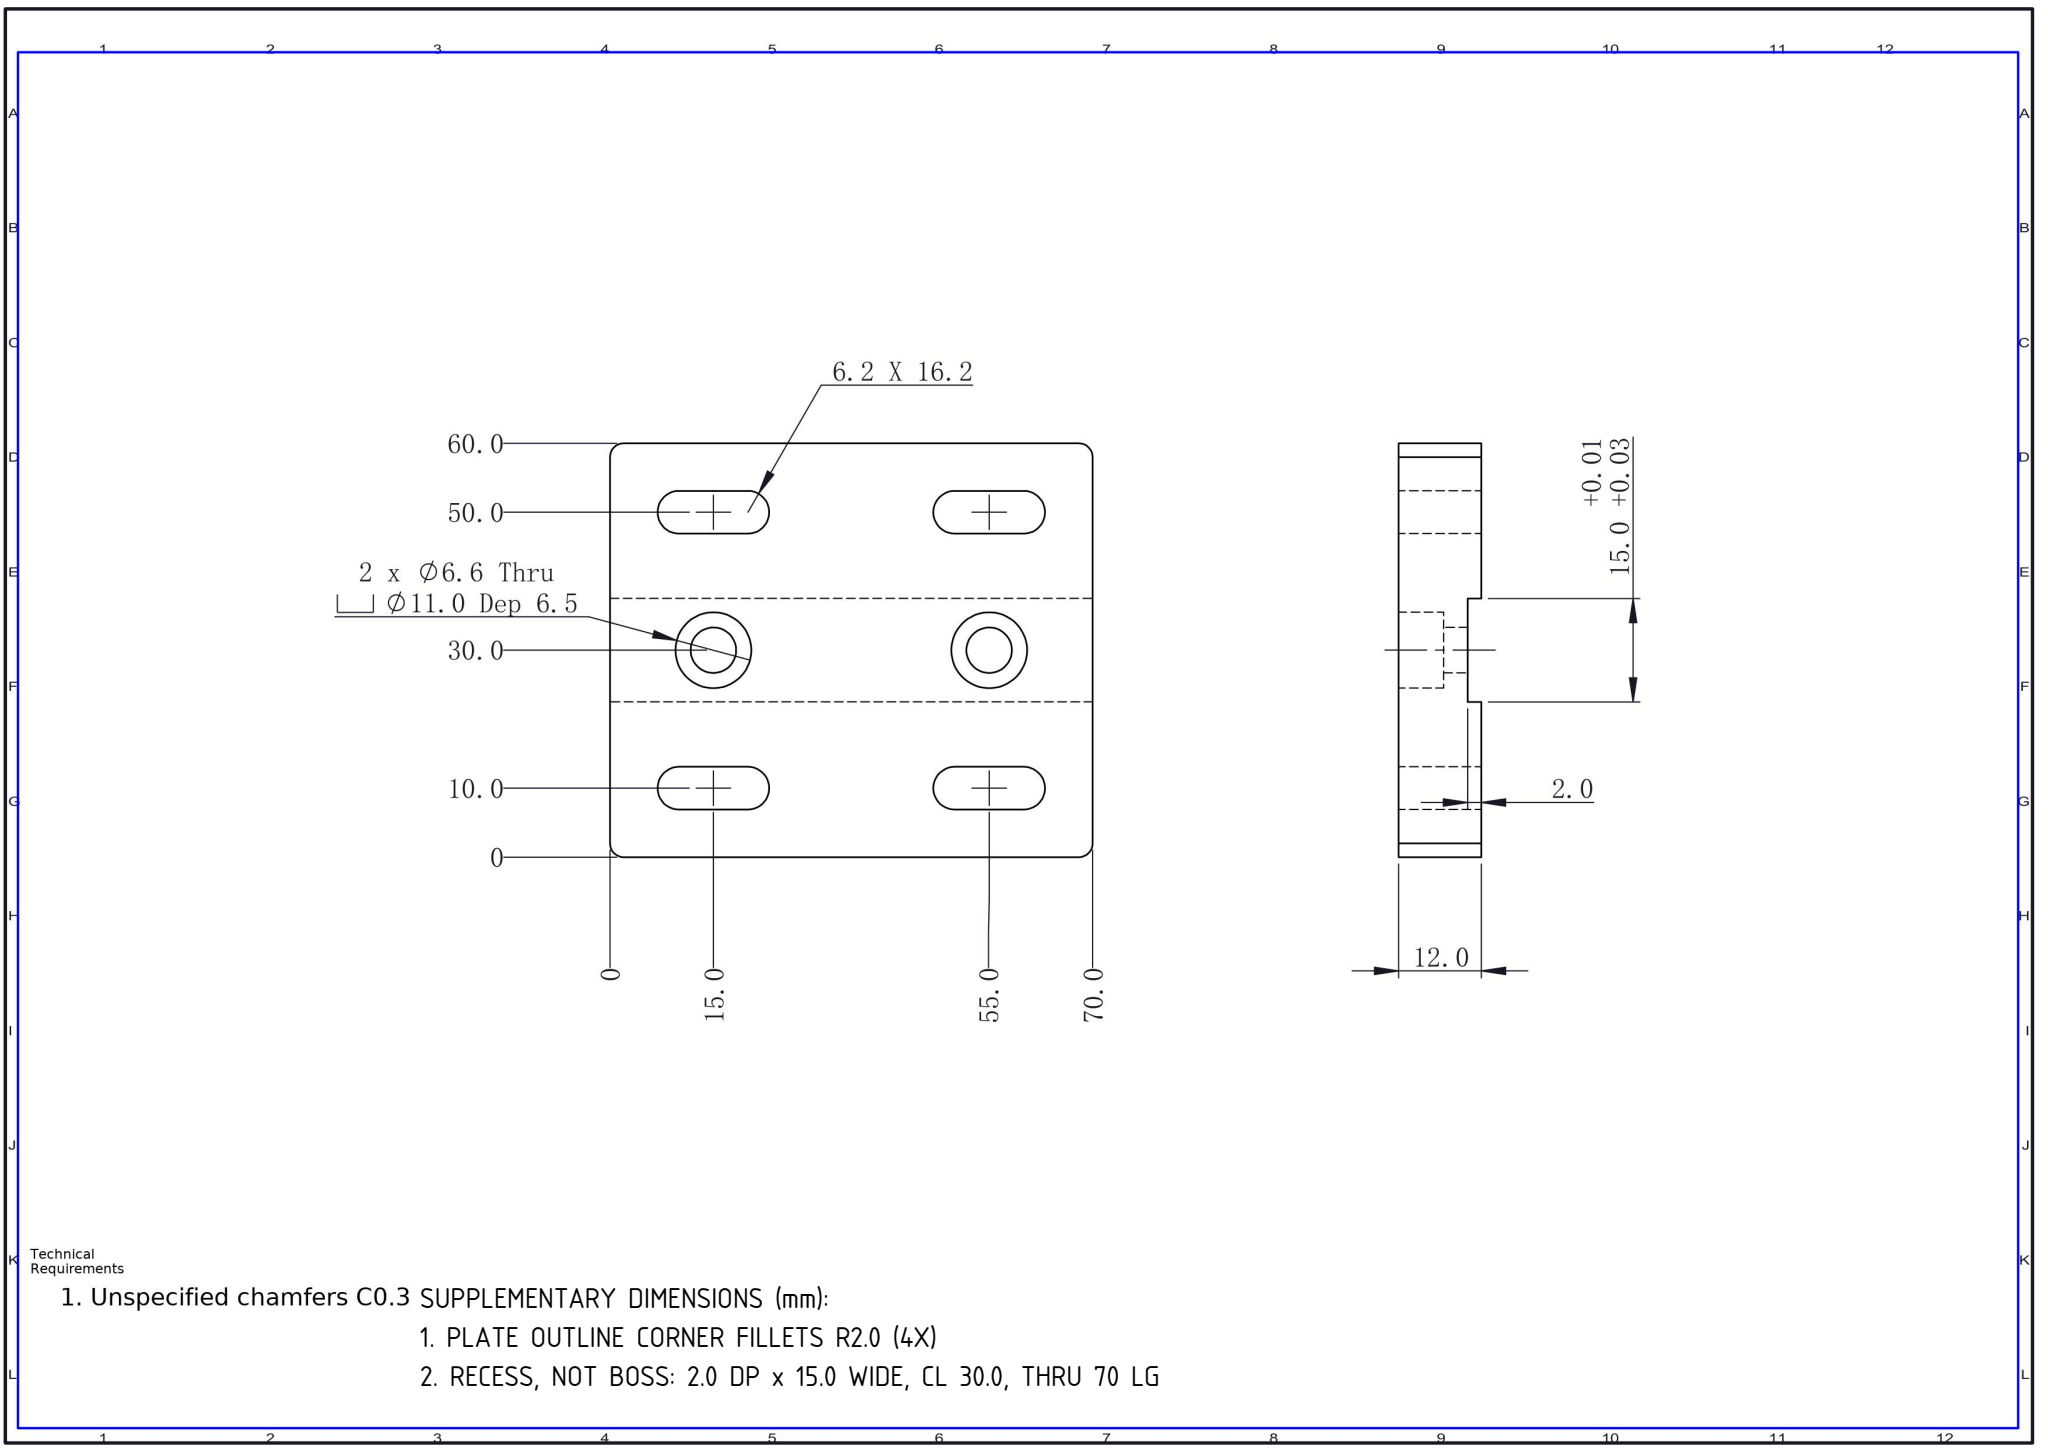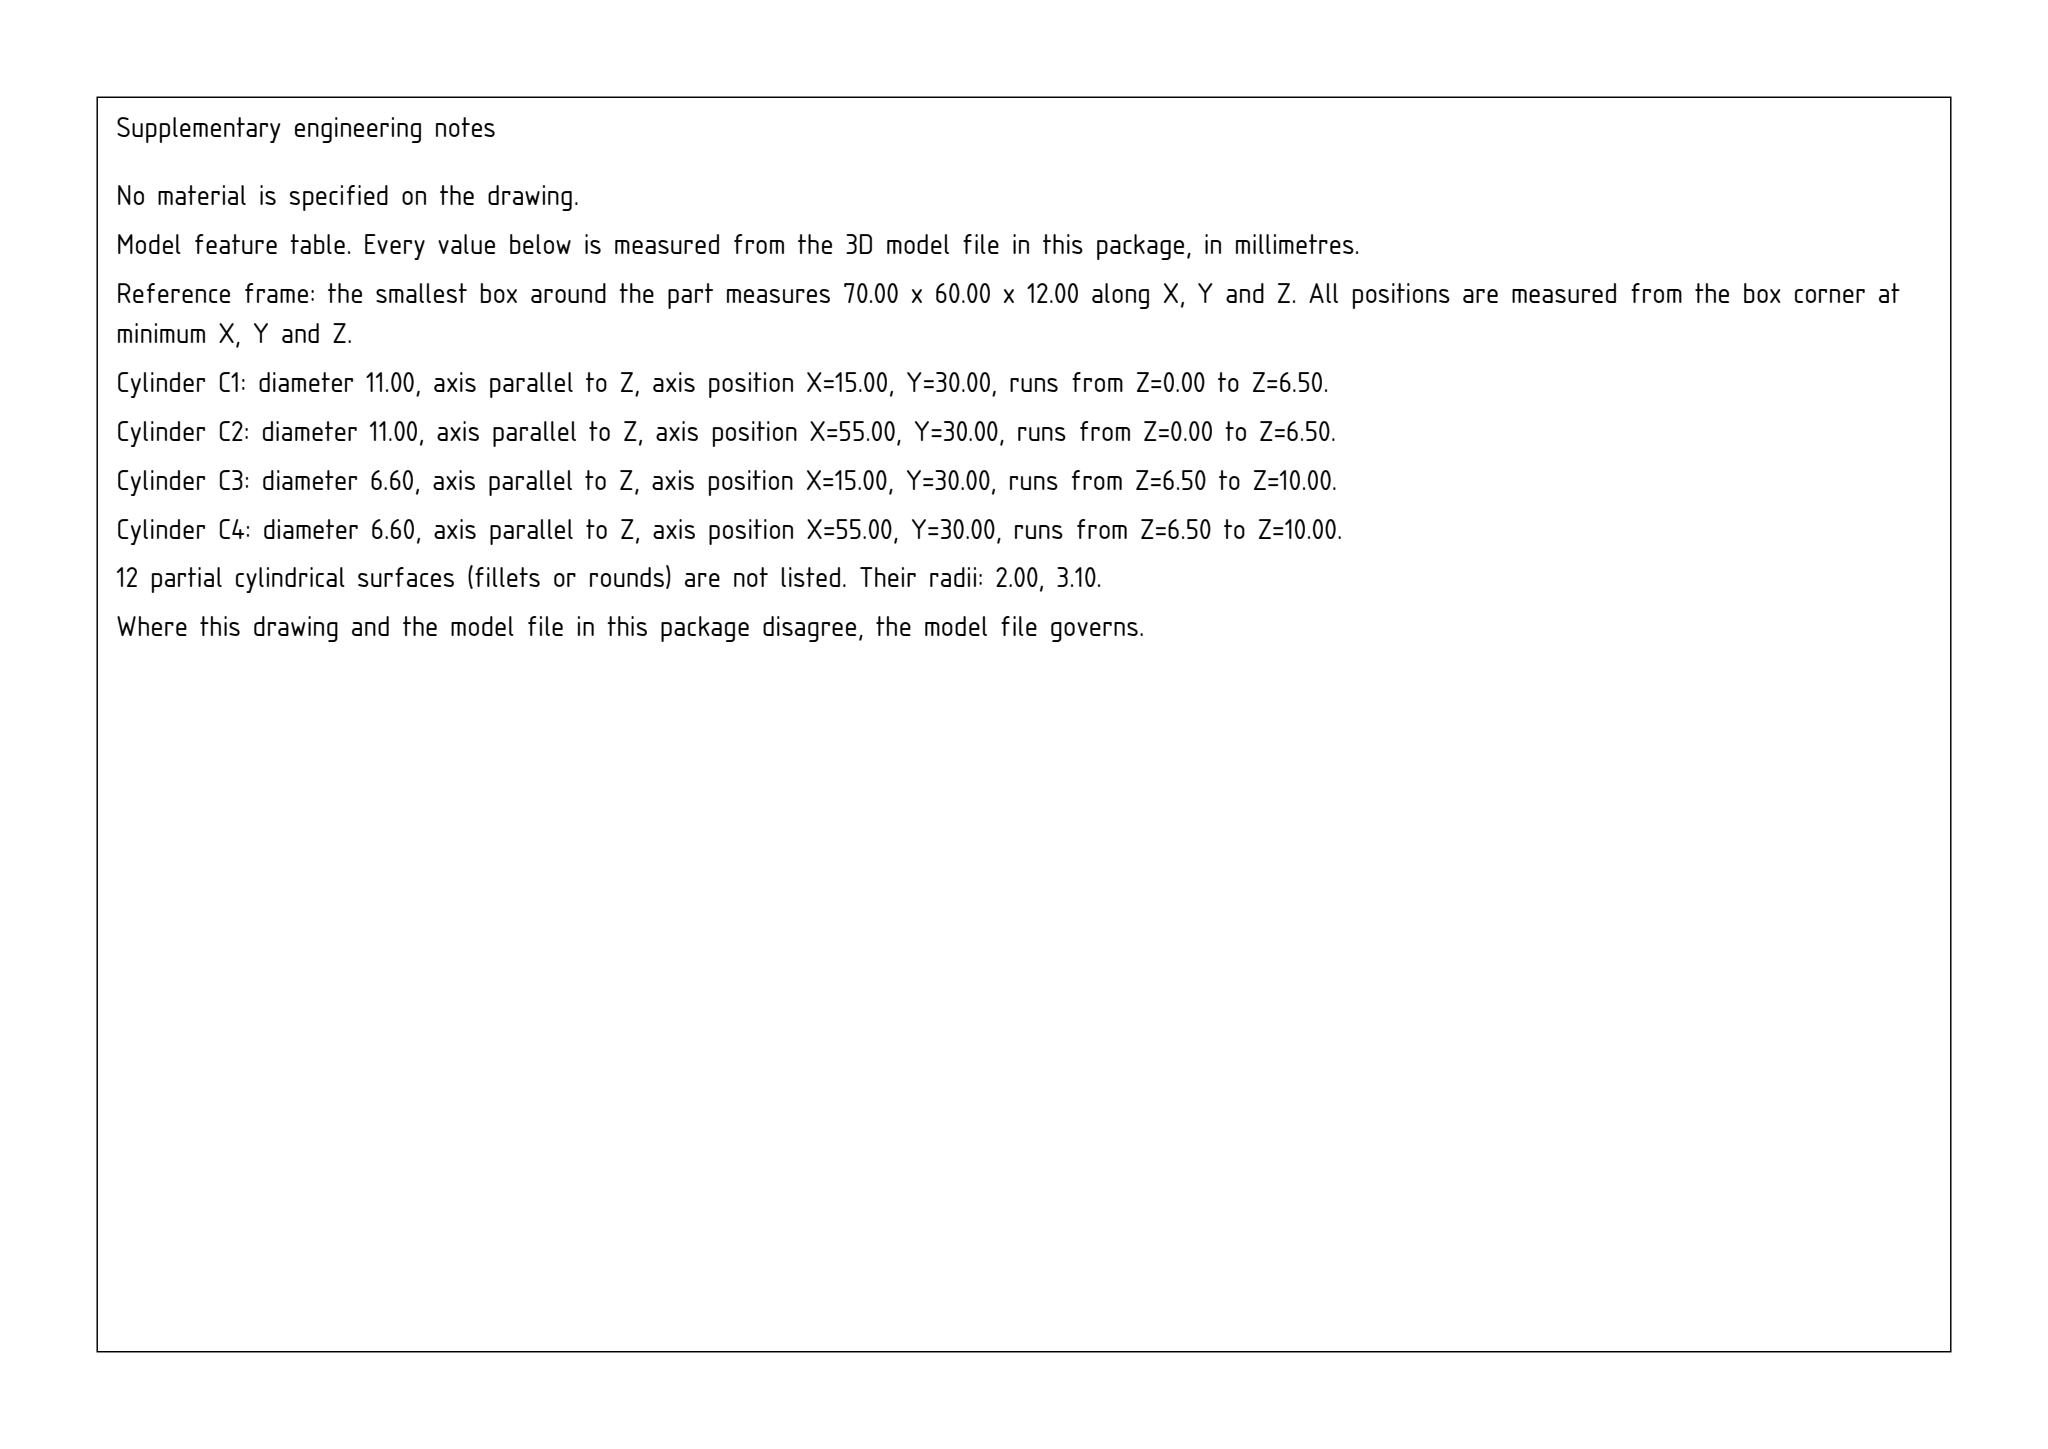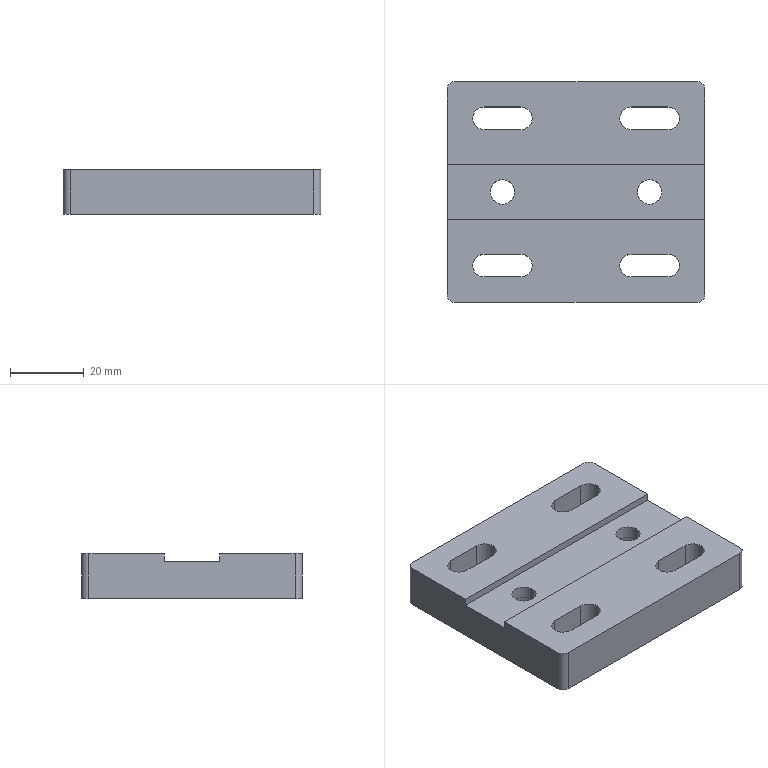Part | SolidWorks | mm | 1 solid | 44 faces | box 70 x 60 x 12 mm | volume 42359 mm3 | cylinder 24 | plane 20 | commonest cylinder face diameters 6.2 x12 11 x4 6.6 x4 4 x4
build123d program:
from build123d import *

# Parameters (mm, degrees)
SKETCH1_W                                       = 70
SKETCH1_H                                       = 60
BOSS_EXTRUDE1_DEPTH                             = 12
SKETCH2_W                                       = 70
SKETCH2_H                                       = 15
CUT_EXTRUDE1_DEPTH                              = 2
FILLET1_R                                       = 2
CUT_EXTRUDE2_DEPTH                              = 48.634
M6_HEX_SOCKET_HEAD_CAP_SCREW_CBORE1_D           = 6.6
M6_HEX_SOCKET_HEAD_CAP_SCREW_CBORE1_CBORE_D     = 11
M6_HEX_SOCKET_HEAD_CAP_SCREW_CBORE1_CBORE_DEPTH = 6.5


with BuildPart() as part:
    # Sketch1 → Boss-Extrude1 (new body)
    with BuildSketch(Plane.XY):
        Rectangle(SKETCH1_W, SKETCH1_H)
    extrude(amount=BOSS_EXTRUDE1_DEPTH)

    # Sketch2 → Cut-Extrude1 (cut)
    with BuildSketch(Plane.XY.offset(12)):
        Rectangle(SKETCH2_W, SKETCH2_H)
    extrude(amount=-CUT_EXTRUDE1_DEPTH, mode=Mode.SUBTRACT)

    # Fillet1
    fillet1_edges = [part.edges().sort_by_distance(p)[0] for p in [
        (35, -30, 6),
        (-35, -30, 6),
        (-35, 30, 6),
        (35, 30, 6),
    ]]
    fillet(fillet1_edges, radius=FILLET1_R)

    # Sketch3 → Cut-Extrude2 (cut, through all)
    with BuildSketch(Plane.XY.offset(12)):
        with BuildLine():
            Line((-25, -16.9), (-15, -16.9))
            ThreePointArc((-15, -16.9), (-11.9, -20), (-15, -23.1))
            Line((-15, -23.1), (-25, -23.1))
            ThreePointArc((-25, -23.1), (-28.1, -20), (-25, -16.9))
        make_face()
        with BuildLine():
            Line((15, -16.9), (25, -16.9))
            ThreePointArc((25, -16.9), (28.1, -20), (25, -23.1))
            Line((25, -23.1), (15, -23.1))
            ThreePointArc((15, -23.1), (11.9, -20), (15, -16.9))
        make_face()
        with BuildLine():
            Line((-25, 23.1), (-15, 23.1))
            ThreePointArc((-15, 23.1), (-11.9, 20), (-15, 16.9))
            Line((-15, 16.9), (-25, 16.9))
            ThreePointArc((-25, 16.9), (-28.1, 20), (-25, 23.1))
        make_face()
        with BuildLine():
            Line((15, 23.1), (25, 23.1))
            ThreePointArc((25, 23.1), (28.1, 20), (25, 16.9))
            Line((25, 16.9), (15, 16.9))
            ThreePointArc((15, 16.9), (11.9, 20), (15, 23.1))
        make_face()
    extrude(amount=-CUT_EXTRUDE2_DEPTH, mode=Mode.SUBTRACT)

    # M6 Hex Socket Head Cap Screw CBORE1 (through all)
    with Locations(Plane(origin=(0, 0, 0), x_dir=(-1, 0, 0), z_dir=(0, 0, -1))):
        with Locations((-20, 0), (20, 0)):
            CounterBoreHole(M6_HEX_SOCKET_HEAD_CAP_SCREW_CBORE1_D / 2, M6_HEX_SOCKET_HEAD_CAP_SCREW_CBORE1_CBORE_D / 2, M6_HEX_SOCKET_HEAD_CAP_SCREW_CBORE1_CBORE_DEPTH)


solid = part.part